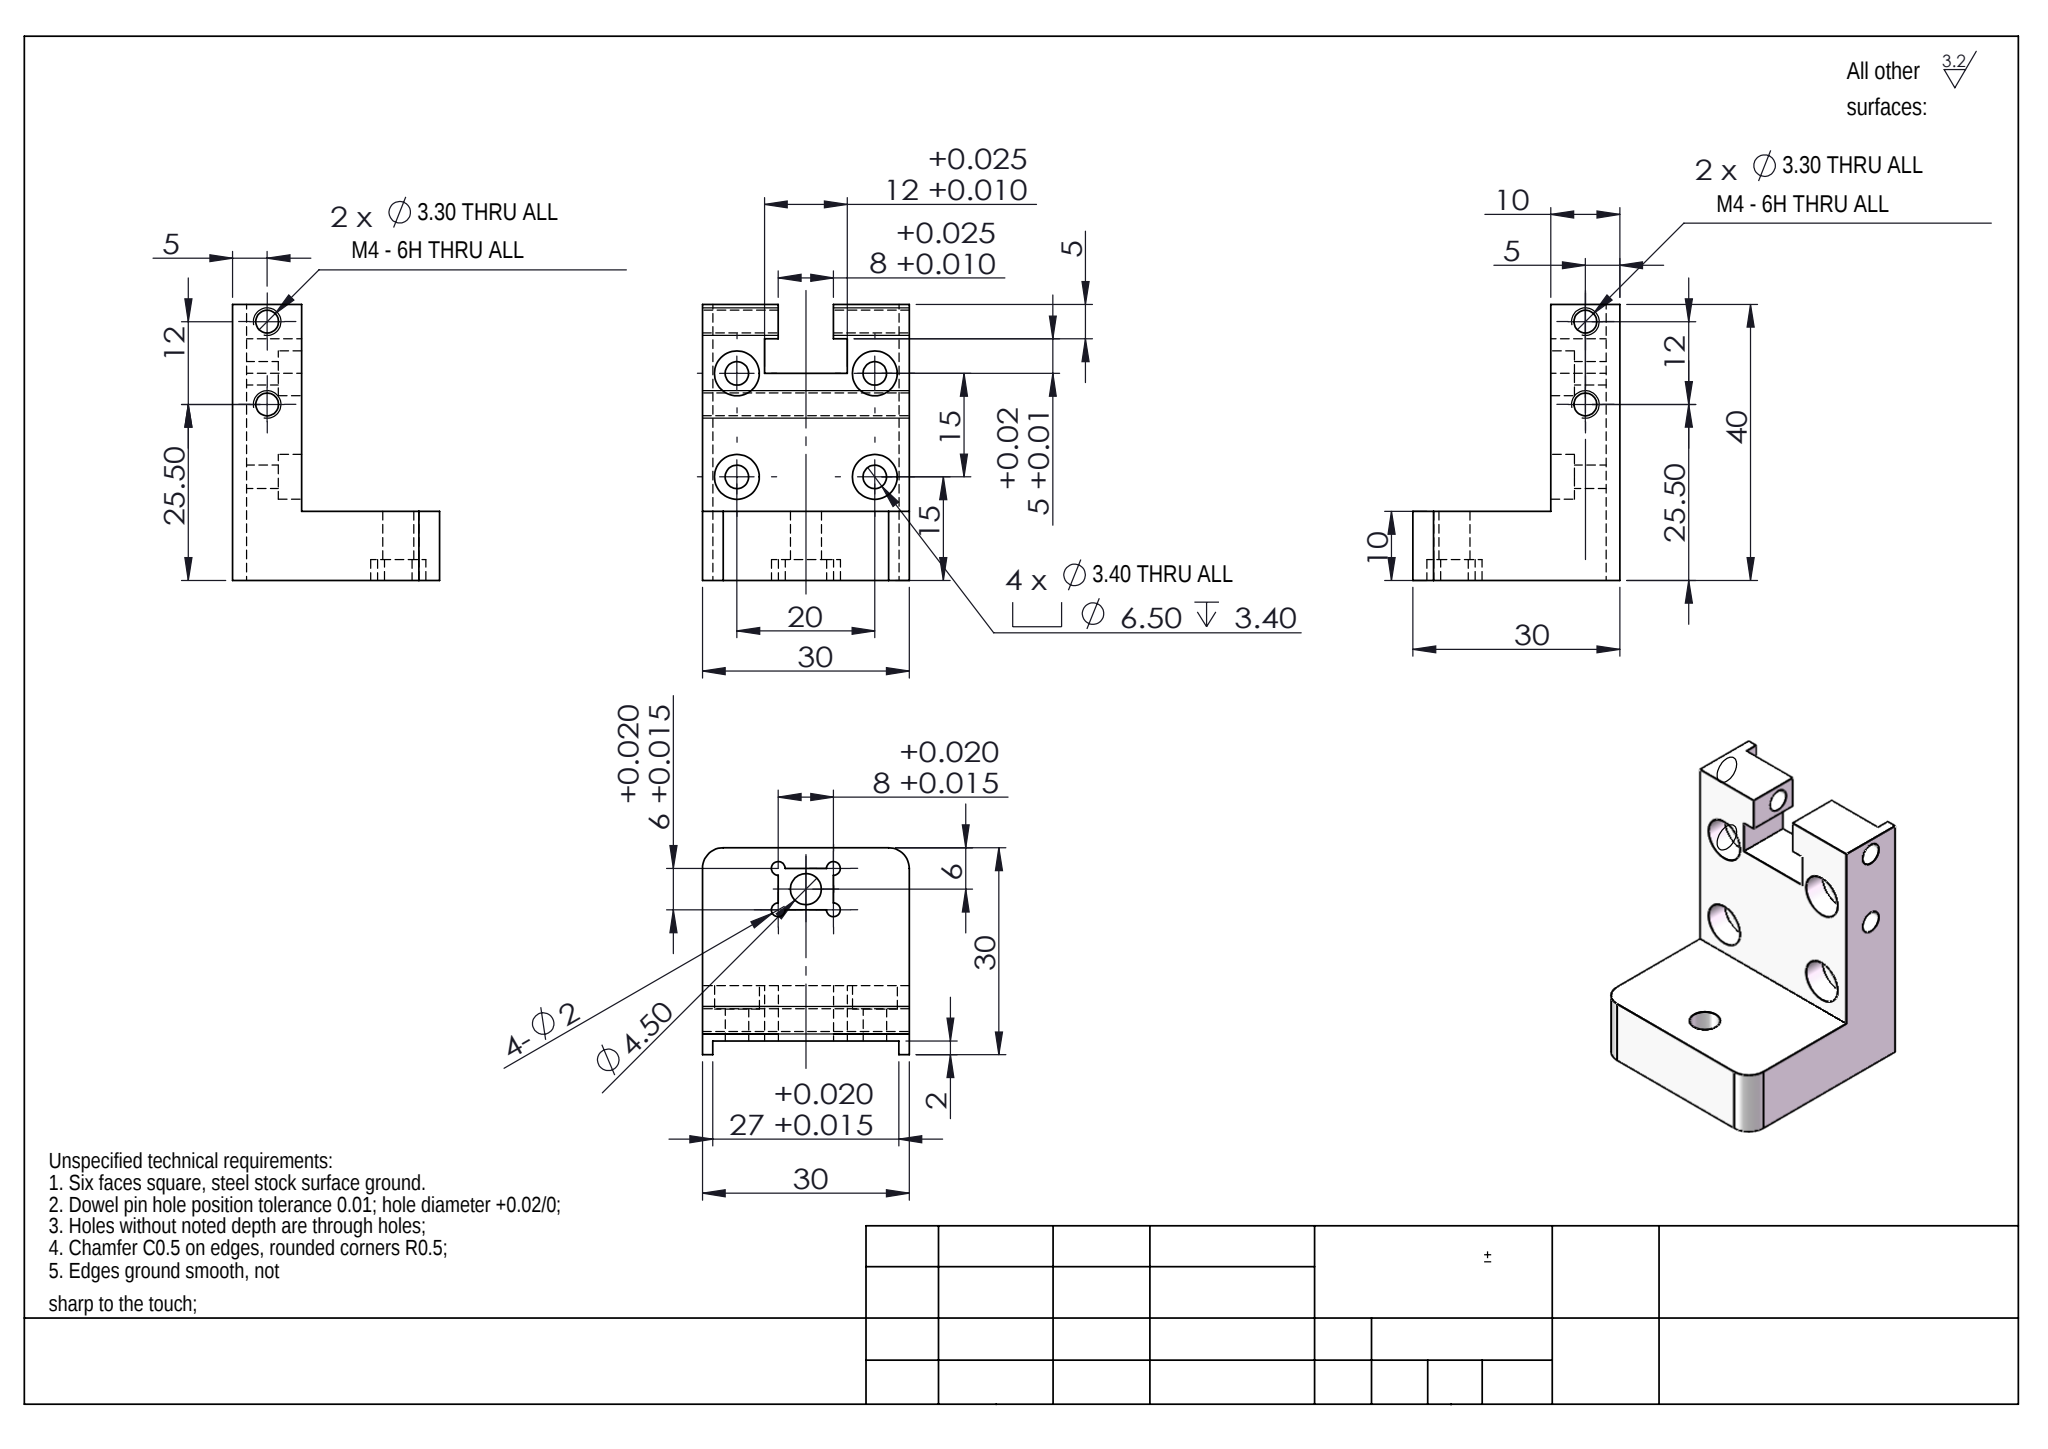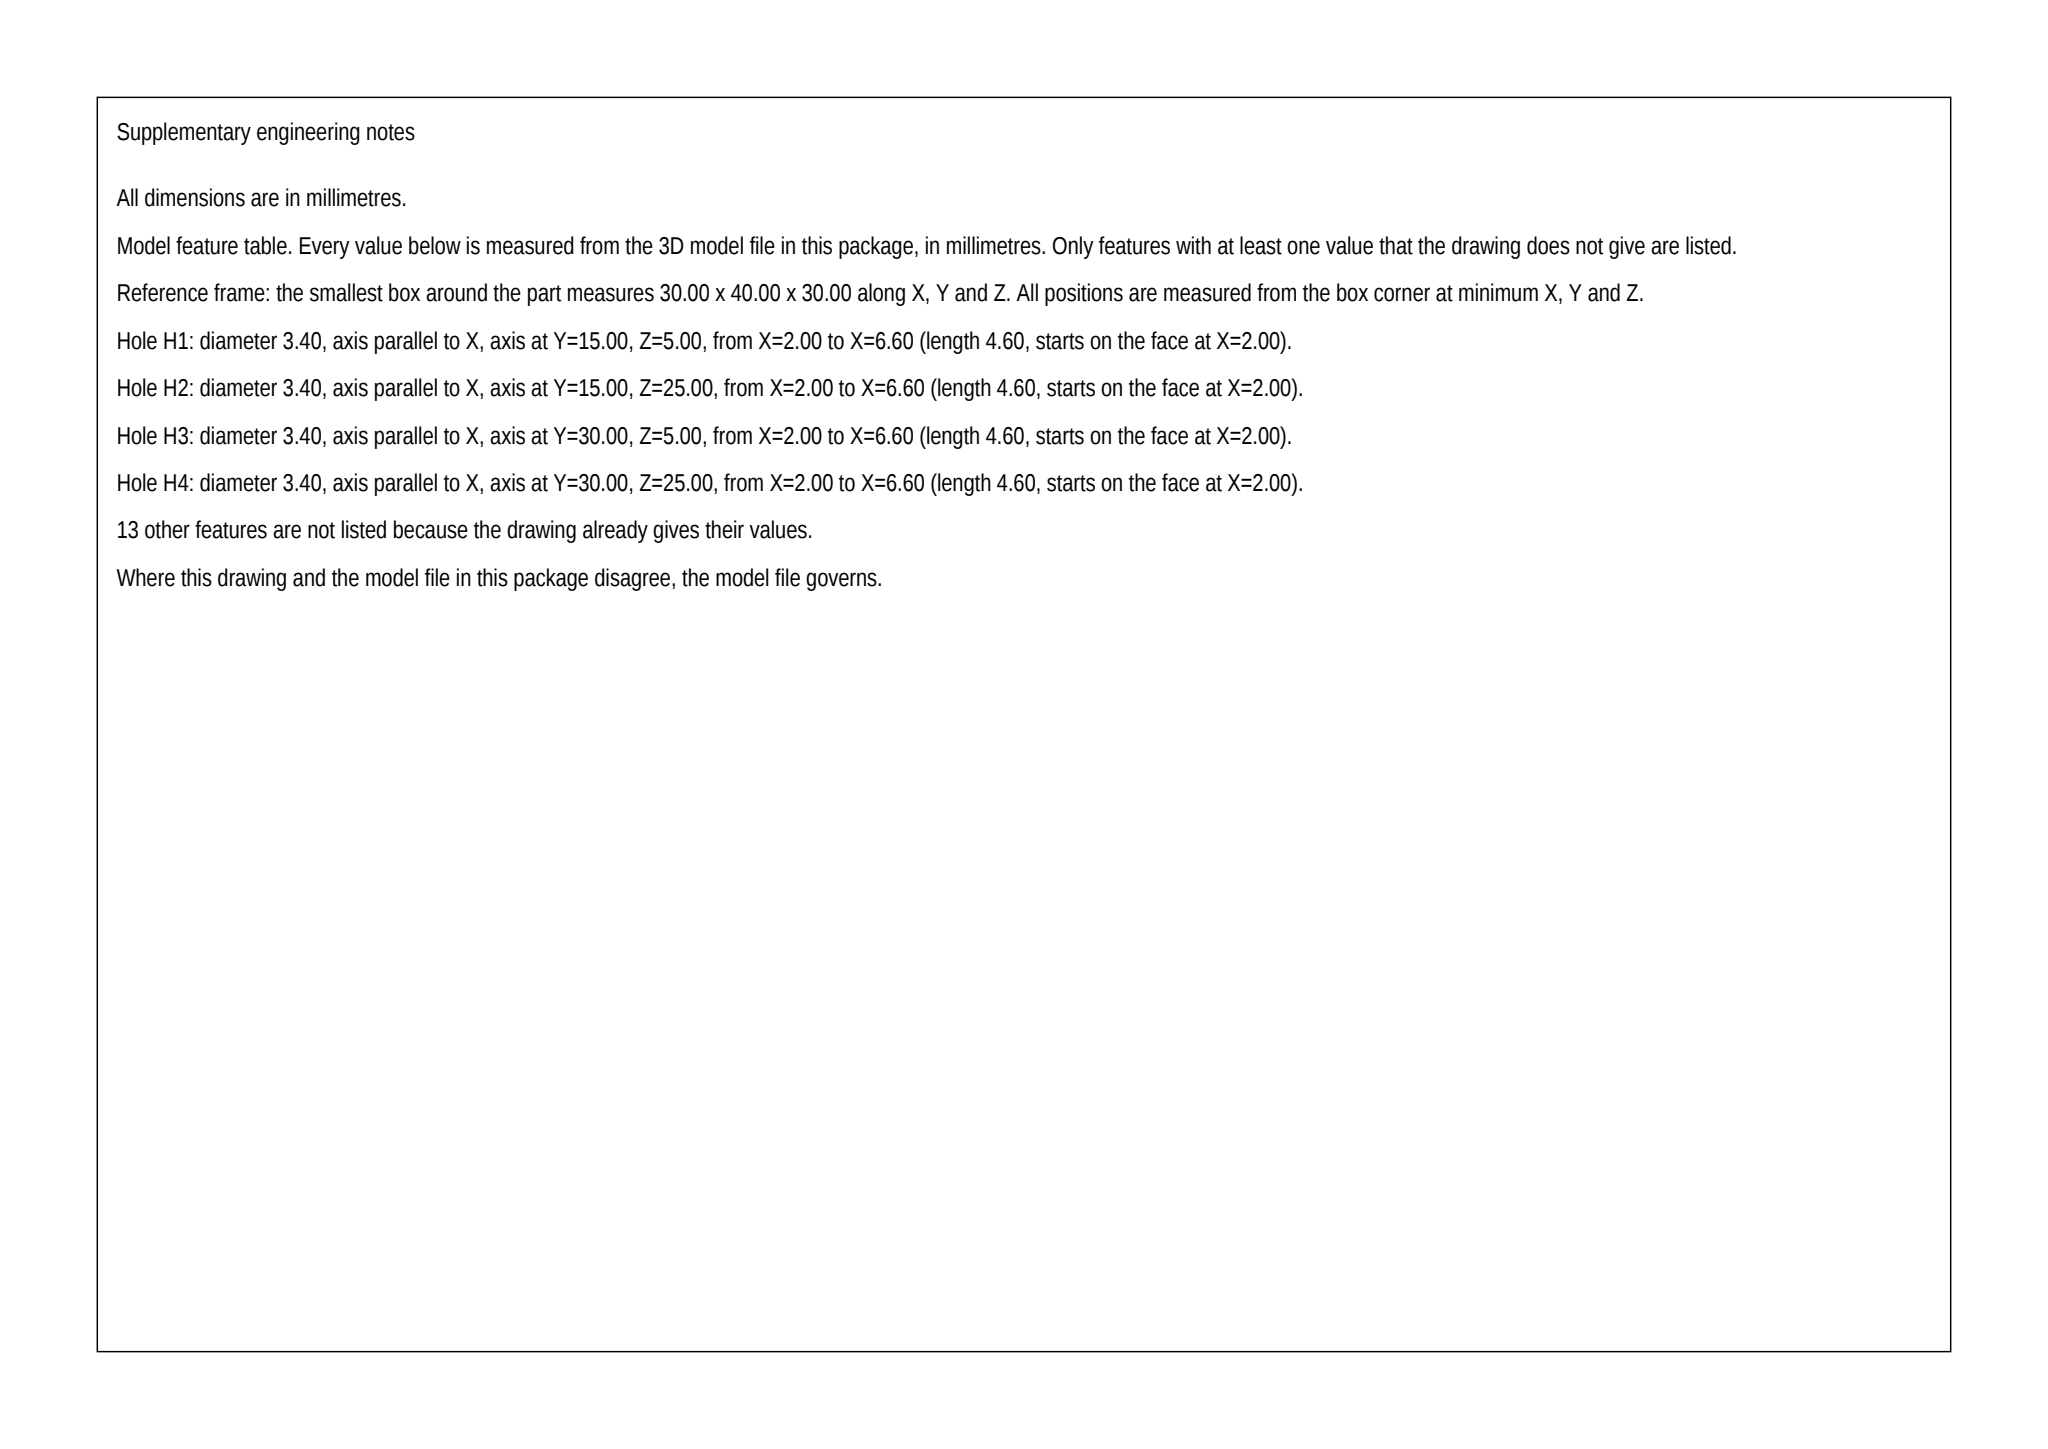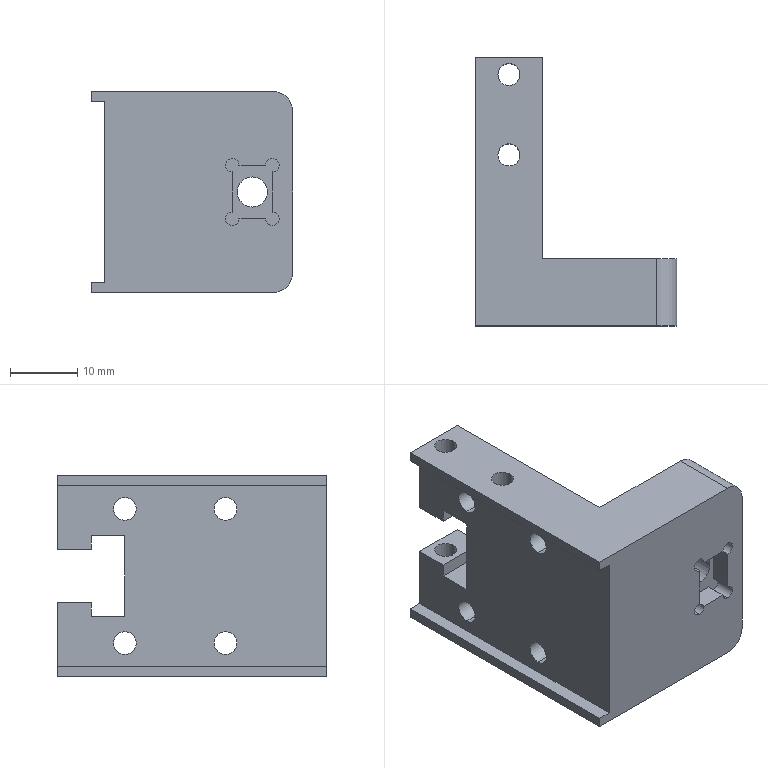Part | SolidWorks | mm | 1 solid | 61 faces | box 30 x 40 x 30 mm | volume 13655 mm3 | cylinder 32 | plane 29 | commonest cylinder face diameters 6.5 x8 3.4 x8 2 x6 3.3 x6 4.5 x2 6 x2
Drawing notes:
BASE PLATE FRONT CORNERS R3 2X, FULL 10 HT | from the solid: Cylinders dia 6.0 axis y at (x=27,z=3) and (x=27,z=27), length 10 = base height y=0-10
TOP SLOT 12 & 8 WIDE SYM ABOUT CL OF 30 WIDTH | from the solid: Planes z=9/21 (12 wide) and z=11/19 (8 wide), both centered on z=15 of 30
UNDERSIDE RELIEF 27 W X 3 DP, 2 FROM BACK FACE THRU FRONT | from the solid: Planes y=3 (recess roof), z=1.5 & 28.5 (27 wide, sym about z=15), x=2 start, open to x=30
build123d program:
from build123d import *

# Parameters (mm, degrees)
SKETCH1_W                                       = 30
SKETCH1_H                                       = 40
BOSS_EXTRUDE1_DEPTH                             = 10
SKETCH2_W                                       = 2
SKETCH2_H                                       = 27
CUT_EXTRUDE1_DEPTH                              = 44.875
SKETCH3_W                                       = 12
SKETCH3_H                                       = 5
CUT_EXTRUDE2_DEPTH                              = 27.926
SKETCH4_W                                       = 8
SKETCH4_H                                       = 5
CUT_EXTRUDE3_DEPTH                              = 27.926
M3_HEX_SOCKET_HEAD_CAP_SCREW_CBORE1_D           = 3.4
M3_HEX_SOCKET_HEAD_CAP_SCREW_CBORE1_CBORE_D     = 6.5
M3_HEX_SOCKET_HEAD_CAP_SCREW_CBORE1_CBORE_DEPTH = 3.4
SKETCH7_W                                       = 30
SKETCH7_H                                       = 10
BOSS_EXTRUDE2_DEPTH                             = 20
M4_TAPPED_HOLE1_D                               = 3.3
SKETCH10_W                                      = 6
SKETCH10_H                                      = 8
CUT_EXTRUDE4_DEPTH                              = 3
SKETCH11_R                                      = 1
CUT_EXTRUDE5_DEPTH                              = 3
SKETCH14_R                                      = 2.25
CUT_EXTRUDE6_DEPTH                              = 10
FILLET1_R                                       = 3


with BuildPart() as part:
    # Sketch1 → Boss-Extrude1 (new body)
    with BuildSketch(Plane(origin=(0, 0, 0), x_dir=(0, 0, -1), z_dir=(1, 0, 0))):
        Rectangle(SKETCH1_W, SKETCH1_H)
    extrude(amount=BOSS_EXTRUDE1_DEPTH)

    # Sketch2 → Cut-Extrude1 (cut, through all)
    with BuildSketch(Plane(origin=(0, 20, 0), x_dir=(1, 0, 0), z_dir=(0, 1, 0))):
        with Locations((1, 0)):
            Rectangle(SKETCH2_W, SKETCH2_H)
    extrude(amount=-CUT_EXTRUDE1_DEPTH, mode=Mode.SUBTRACT)

    # Sketch3 → Cut-Extrude2 (cut, through all)
    with BuildSketch(Plane(origin=(10, 0, 0), x_dir=(0, 0, -1), z_dir=(1, 0, 0))):
        with Locations((0, 12.5)):
            Rectangle(SKETCH3_W, SKETCH3_H)
    extrude(amount=-CUT_EXTRUDE2_DEPTH, mode=Mode.SUBTRACT)

    # Sketch4 → Cut-Extrude3 (cut, through all)
    with BuildSketch(Plane(origin=(10, 0, 0), x_dir=(0, 0, -1), z_dir=(1, 0, 0))):
        with Locations((0, 17.5)):
            Rectangle(SKETCH4_W, SKETCH4_H)
    extrude(amount=-CUT_EXTRUDE3_DEPTH, mode=Mode.SUBTRACT)

    # M3 Hex Socket Head Cap Screw CBORE1 (through all)
    with Locations(Plane(origin=(10, 0, 0), x_dir=(0, 0, -1), z_dir=(1, 0, 0))):
        with Locations((-10, 10), (10, 10), (-10, -5), (10, -5)):
            CounterBoreHole(M3_HEX_SOCKET_HEAD_CAP_SCREW_CBORE1_D / 2, M3_HEX_SOCKET_HEAD_CAP_SCREW_CBORE1_CBORE_D / 2, M3_HEX_SOCKET_HEAD_CAP_SCREW_CBORE1_CBORE_DEPTH)

    # Sketch7 → Boss-Extrude2 (add)
    with BuildSketch(Plane(origin=(10, 0, 0), x_dir=(0, 0, -1), z_dir=(1, 0, 0))):
        with Locations((0, -15)):
            Rectangle(SKETCH7_W, SKETCH7_H)
    extrude(amount=BOSS_EXTRUDE2_DEPTH)

    # M4 Tapped Hole1 (through all)
    with Locations(Plane.XY.offset(15)):
        with Locations((5, 5.5), (5, 17.5)):
            Hole(M4_TAPPED_HOLE1_D / 2)

    # Sketch10 → Cut-Extrude4 (cut)
    with BuildSketch(Plane.XZ.offset(20)):
        with Locations((24, 0)):
            Rectangle(SKETCH10_W, SKETCH10_H)
    extrude(amount=-CUT_EXTRUDE4_DEPTH, mode=Mode.SUBTRACT)

    # Sketch11 → Cut-Extrude5 (cut)
    with BuildSketch(Plane.XZ.offset(20)):
        with Locations((21, 4)):
            Circle(SKETCH11_R)
        with Locations((27, 4)):
            Circle(SKETCH11_R)
        with Locations((21, -4)):
            Circle(SKETCH11_R)
        with Locations((27, -4)):
            Circle(SKETCH11_R)
    extrude(amount=-CUT_EXTRUDE5_DEPTH, mode=Mode.SUBTRACT)

    # Sketch14 → Cut-Extrude6 (cut)
    with BuildSketch(Plane(origin=(0, -10, 0), x_dir=(1, 0, 0), z_dir=(0, 1, 0))):
        with Locations(Location((24, 0, 0), (0, 0, 270))):
            Circle(SKETCH14_R)
    extrude(amount=-CUT_EXTRUDE6_DEPTH, mode=Mode.SUBTRACT)

    # Fillet1
    fillet1_edges = [part.edges().sort_by_distance(p)[0] for p in [
        (30, -15, 15),
        (30, -15, -15),
    ]]
    fillet(fillet1_edges, radius=FILLET1_R)


solid = part.part